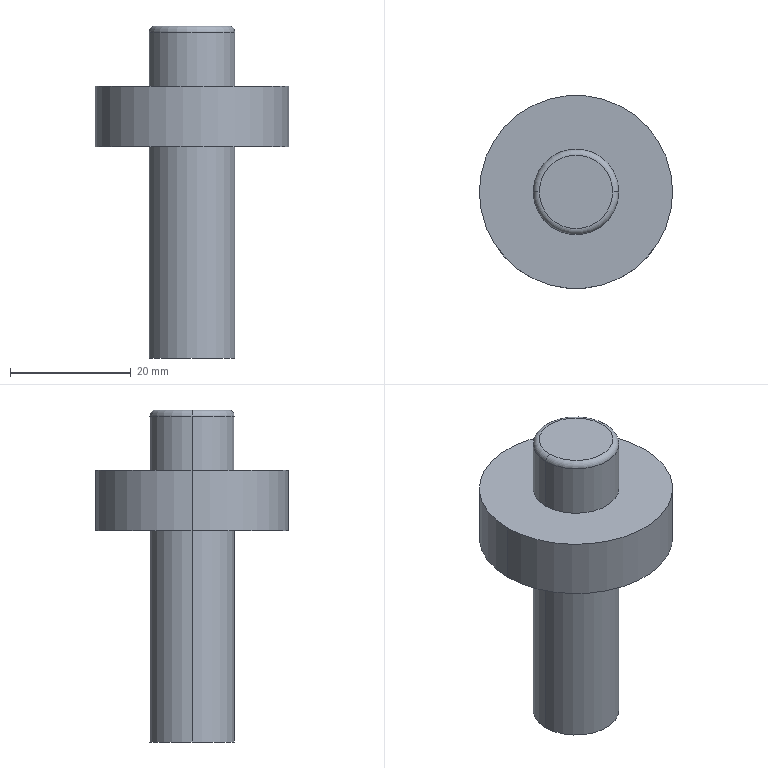Component | SolidWorks | Motor-1 | 1 solid | 12 faces | box 32.01 x 32.01 x 55 mm | volume 15143 mm3 | cylinder 6 | plane 4 | torus 2 | commonest cylinder face diameters 14.18 x4 32.008 x2
build123d program:
from build123d import *

# Parameters (mm, degrees)
SKETCH1_R           = 16.004
BOSS_EXTRUDE1_DEPTH = 10
SKETCH2_R           = 7.09
BOSS_EXTRUDE2_DEPTH = 10
FILLET1_R           = 1
BOSS_EXTRUDE3_START = 35
SKETCH3_R           = 7.09
BOSS_EXTRUDE3_DEPTH = 35


with BuildPart() as part:
    # Sketch1 → Boss-Extrude1 (new body)
    with BuildSketch(Plane.XY):
        with Locations((209.842, -12.569)):
            Circle(SKETCH1_R)
    extrude(amount=BOSS_EXTRUDE1_DEPTH)

    # Sketch2 → Boss-Extrude2 (add)
    with BuildSketch(Plane.XY.offset(10)):
        with Locations((209.842, -12.569)):
            Circle(SKETCH2_R)
    extrude(amount=BOSS_EXTRUDE2_DEPTH)

    # Fillet1
    fillet1_edges = [part.edges().sort_by_distance(p)[0] for p in [
        (202.752, -12.569, 20),
    ]]
    fillet(fillet1_edges, radius=FILLET1_R)

    # Sketch3 → Boss-Extrude3 (add)
    with BuildSketch(Plane(origin=(0, 0, 0), x_dir=(-1, 0, 0), z_dir=(0, 0, -1)).offset(BOSS_EXTRUDE3_START)):
        with Locations(Location((-209.842, -12.569, 0), (0, 0, 180))):
            Circle(SKETCH3_R)
    extrude(amount=-BOSS_EXTRUDE3_DEPTH)


solid = part.part

# Placed as in the assembly
solid = solid.moved(Location((-16.965, 0.5467, 8.5), (0, 0, 0)))
STEP:
#1=COLOUR_RGB('',0.7922,0.8196,0.9333);
#2=FILL_AREA_STYLE_COLOUR('',#1);
#3=FILL_AREA_STYLE('',(#2));
#4=SURFACE_STYLE_FILL_AREA(#3);
#5=SURFACE_SIDE_STYLE('',(#4));
#6=SURFACE_STYLE_USAGE(.BOTH.,#5);
#7=PRESENTATION_STYLE_ASSIGNMENT((#6));
#8=CARTESIAN_POINT('',(7.314,-0.4733,-1.043));
#9=VERTEX_POINT('',#8);
#10=CARTESIAN_POINT('',(7.873,-0.4733,-1.043));
#11=VERTEX_POINT('',#10);
#12=CARTESIAN_POINT('',(7.594,-0.4733,-1.043));
#13=DIRECTION('',(0.,0.,-1.));
#14=DIRECTION('',(-1.,0.,0.));
#15=AXIS2_PLACEMENT_3D('',#12,#13,#14);
#16=CIRCLE('',#15,0.2791);
#17=EDGE_CURVE('',#9,#11,#16,.T.);
#18=ORIENTED_EDGE('',*,*,#17,.F.);
#19=CARTESIAN_POINT('',(7.314,-0.4733,0.3346));
#20=VERTEX_POINT('',#19);
#21=CARTESIAN_POINT('',(7.314,-0.4733,-1.043));
#22=DIRECTION('',(0.,0.,1.));
#23=VECTOR('',#22,39.37);
#24=LINE('',#21,#23);
#25=EDGE_CURVE('',#9,#20,#24,.T.);
#26=ORIENTED_EDGE('',*,*,#25,.T.);
#27=CARTESIAN_POINT('',(7.873,-0.4733,0.3346));
#28=VERTEX_POINT('',#27);
#29=CARTESIAN_POINT('',(7.594,-0.4733,0.3346));
#30=DIRECTION('',(0.,0.,-1.));
#31=DIRECTION('',(-1.,0.,0.));
#32=AXIS2_PLACEMENT_3D('',#29,#30,#31);
#33=CIRCLE('',#32,0.2791);
#34=EDGE_CURVE('',#20,#28,#33,.T.);
#35=ORIENTED_EDGE('',*,*,#34,.T.);
#36=CARTESIAN_POINT('',(7.873,-0.4733,-1.043));
#37=DIRECTION('',(0.,0.,1.));
#38=VECTOR('',#37,39.37);
#39=LINE('',#36,#38);
#40=EDGE_CURVE('',#11,#28,#39,.T.);
#41=ORIENTED_EDGE('',*,*,#40,.F.);
#42=EDGE_LOOP('',(#18,#26,#35,#41));
#43=FACE_OUTER_BOUND('',#42,.T.);
#44=CARTESIAN_POINT('',(7.594,-0.4733,-1.043));
#45=DIRECTION('',(0.,0.,1.));
#46=DIRECTION('',(1.,0.,0.));
#47=AXIS2_PLACEMENT_3D('',#44,#45,#46);
#48=CYLINDRICAL_SURFACE('',#47,0.2791);
#49=ADVANCED_FACE('',(#43),#48,.T.);
#50=CARTESIAN_POINT('',(7.314,-0.4733,1.083));
#51=VERTEX_POINT('',#50);
#52=CARTESIAN_POINT('',(7.873,-0.4733,1.083));
#53=VERTEX_POINT('',#52);
#54=CARTESIAN_POINT('',(7.594,-0.4733,1.083));
#55=DIRECTION('',(0.,0.,-1.));
#56=DIRECTION('',(1.,0.,0.));
#57=AXIS2_PLACEMENT_3D('',#54,#55,#56);
#58=CIRCLE('',#57,0.2791);
#59=EDGE_CURVE('',#51,#53,#58,.T.);
#60=ORIENTED_EDGE('',*,*,#59,.F.);
#61=CARTESIAN_POINT('',(7.354,-0.4733,1.122));
#62=VERTEX_POINT('',#61);
#63=CARTESIAN_POINT('',(7.354,-0.4733,1.083));
#64=DIRECTION('',(0.,1.,0.));
#65=DIRECTION('',(-1.,0.,0.));
#66=AXIS2_PLACEMENT_3D('',#63,#64,#65);
#67=CIRCLE('',#66,0.03937);
#68=EDGE_CURVE('',#51,#62,#67,.T.);
#69=ORIENTED_EDGE('',*,*,#68,.T.);
#70=CARTESIAN_POINT('',(7.833,-0.4733,1.122));
#71=VERTEX_POINT('',#70);
#72=CARTESIAN_POINT('',(7.594,-0.4733,1.122));
#73=DIRECTION('',(0.,0.,1.));
#74=DIRECTION('',(1.,0.,0.));
#75=AXIS2_PLACEMENT_3D('',#72,#73,#74);
#76=CIRCLE('',#75,0.2398);
#77=EDGE_CURVE('',#71,#62,#76,.T.);
#78=ORIENTED_EDGE('',*,*,#77,.F.);
#79=CARTESIAN_POINT('',(7.833,-0.4733,1.083));
#80=DIRECTION('',(0.,-1.,0.));
#81=DIRECTION('',(0.,0.,-1.));
#82=AXIS2_PLACEMENT_3D('',#79,#80,#81);
#83=CIRCLE('',#82,0.03937);
#84=EDGE_CURVE('',#53,#71,#83,.T.);
#85=ORIENTED_EDGE('',*,*,#84,.F.);
#86=EDGE_LOOP('',(#60,#69,#78,#85));
#87=FACE_OUTER_BOUND('',#86,.T.);
#88=CARTESIAN_POINT('',(7.594,-0.4733,1.083));
#89=DIRECTION('',(0.,0.,1.));
#90=DIRECTION('',(1.,0.,0.));
#91=AXIS2_PLACEMENT_3D('',#88,#89,#90);
#92=TOROIDAL_SURFACE('',#91,0.2398,0.03937);
#93=ADVANCED_FACE('',(#87),#92,.T.);
#94=ORIENTED_EDGE('',*,*,#59,.T.);
#95=CARTESIAN_POINT('',(7.873,-0.4733,0.7283));
#96=VERTEX_POINT('',#95);
#97=CARTESIAN_POINT('',(7.873,-0.4733,1.122));
#98=DIRECTION('',(0.,0.,-1.));
#99=VECTOR('',#98,39.37);
#100=LINE('',#97,#99);
#101=EDGE_CURVE('',#53,#96,#100,.T.);
#102=ORIENTED_EDGE('',*,*,#101,.T.);
#103=CARTESIAN_POINT('',(7.314,-0.4733,0.7283));
#104=VERTEX_POINT('',#103);
#105=CARTESIAN_POINT('',(7.594,-0.4733,0.7283));
#106=DIRECTION('',(0.,0.,1.));
#107=DIRECTION('',(1.,0.,0.));
#108=AXIS2_PLACEMENT_3D('',#105,#106,#107);
#109=CIRCLE('',#108,0.2791);
#110=EDGE_CURVE('',#96,#104,#109,.T.);
#111=ORIENTED_EDGE('',*,*,#110,.T.);
#112=CARTESIAN_POINT('',(7.314,-0.4733,1.122));
#113=DIRECTION('',(0.,0.,-1.));
#114=VECTOR('',#113,39.37);
#115=LINE('',#112,#114);
#116=EDGE_CURVE('',#51,#104,#115,.T.);
#117=ORIENTED_EDGE('',*,*,#116,.F.);
#118=EDGE_LOOP('',(#94,#102,#111,#117));
#119=FACE_OUTER_BOUND('',#118,.T.);
#120=CARTESIAN_POINT('',(7.594,-0.4733,1.122));
#121=DIRECTION('',(0.,0.,-1.));
#122=DIRECTION('',(-1.,0.,0.));
#123=AXIS2_PLACEMENT_3D('',#120,#121,#122);
#124=CYLINDRICAL_SURFACE('',#123,0.2791);
#125=ADVANCED_FACE('',(#119),#124,.T.);
#126=CARTESIAN_POINT('',(8.224,-0.4733,0.7283));
#127=VERTEX_POINT('',#126);
#128=CARTESIAN_POINT('',(6.964,-0.4733,0.7283));
#129=VERTEX_POINT('',#128);
#130=CARTESIAN_POINT('',(7.594,-0.4733,0.7283));
#131=DIRECTION('',(0.,0.,1.));
#132=DIRECTION('',(1.,0.,0.));
#133=AXIS2_PLACEMENT_3D('',#130,#131,#132);
#134=CIRCLE('',#133,0.6301);
#135=EDGE_CURVE('',#127,#129,#134,.T.);
#136=ORIENTED_EDGE('',*,*,#135,.F.);
#137=CARTESIAN_POINT('',(8.224,-0.4733,0.3346));
#138=VERTEX_POINT('',#137);
#139=CARTESIAN_POINT('',(8.224,-0.4733,0.7283));
#140=DIRECTION('',(0.,0.,-1.));
#141=VECTOR('',#140,39.37);
#142=LINE('',#139,#141);
#143=EDGE_CURVE('',#127,#138,#142,.T.);
#144=ORIENTED_EDGE('',*,*,#143,.T.);
#145=CARTESIAN_POINT('',(6.964,-0.4733,0.3346));
#146=VERTEX_POINT('',#145);
#147=CARTESIAN_POINT('',(7.594,-0.4733,0.3346));
#148=DIRECTION('',(0.,0.,1.));
#149=DIRECTION('',(1.,0.,0.));
#150=AXIS2_PLACEMENT_3D('',#147,#148,#149);
#151=CIRCLE('',#150,0.6301);
#152=EDGE_CURVE('',#138,#146,#151,.T.);
#153=ORIENTED_EDGE('',*,*,#152,.T.);
#154=CARTESIAN_POINT('',(6.964,-0.4733,0.7283));
#155=DIRECTION('',(0.,0.,-1.));
#156=VECTOR('',#155,39.37);
#157=LINE('',#154,#156);
#158=EDGE_CURVE('',#129,#146,#157,.T.);
#159=ORIENTED_EDGE('',*,*,#158,.F.);
#160=EDGE_LOOP('',(#136,#144,#153,#159));
#161=FACE_OUTER_BOUND('',#160,.T.);
#162=CARTESIAN_POINT('',(7.594,-0.4733,0.7283));
#163=DIRECTION('',(0.,0.,-1.));
#164=DIRECTION('',(-1.,0.,0.));
#165=AXIS2_PLACEMENT_3D('',#162,#163,#164);
#166=CYLINDRICAL_SURFACE('',#165,0.6301);
#167=ADVANCED_FACE('',(#161),#166,.T.);
#168=ORIENTED_EDGE('',*,*,#143,.F.);
#169=CARTESIAN_POINT('',(7.594,-0.4733,0.7283));
#170=DIRECTION('',(0.,0.,1.));
#171=DIRECTION('',(1.,0.,0.));
#172=AXIS2_PLACEMENT_3D('',#169,#170,#171);
#173=CIRCLE('',#172,0.6301);
#174=EDGE_CURVE('',#129,#127,#173,.T.);
#175=ORIENTED_EDGE('',*,*,#174,.F.);
#176=ORIENTED_EDGE('',*,*,#158,.T.);
#177=CARTESIAN_POINT('',(7.594,-0.4733,0.3346));
#178=DIRECTION('',(0.,0.,1.));
#179=DIRECTION('',(1.,0.,0.));
#180=AXIS2_PLACEMENT_3D('',#177,#178,#179);
#181=CIRCLE('',#180,0.6301);
#182=EDGE_CURVE('',#146,#138,#181,.T.);
#183=ORIENTED_EDGE('',*,*,#182,.T.);
#184=EDGE_LOOP('',(#168,#175,#176,#183));
#185=FACE_OUTER_BOUND('',#184,.T.);
#186=CARTESIAN_POINT('',(7.594,-0.4733,0.7283));
#187=DIRECTION('',(0.,0.,-1.));
#188=DIRECTION('',(-1.,0.,0.));
#189=AXIS2_PLACEMENT_3D('',#186,#187,#188);
#190=CYLINDRICAL_SURFACE('',#189,0.6301);
#191=ADVANCED_FACE('',(#185),#190,.T.);
#192=CARTESIAN_POINT('',(7.594,-0.4733,0.7283));
#193=DIRECTION('',(0.,0.,1.));
#194=DIRECTION('',(1.,0.,0.));
#195=AXIS2_PLACEMENT_3D('',#192,#193,#194);
#196=CIRCLE('',#195,0.2791);
#197=EDGE_CURVE('',#104,#96,#196,.T.);
#198=ORIENTED_EDGE('',*,*,#197,.F.);
#199=ORIENTED_EDGE('',*,*,#110,.F.);
#200=EDGE_LOOP('',(#198,#199));
#201=FACE_BOUND('',#200,.T.);
#202=ORIENTED_EDGE('',*,*,#174,.T.);
#203=ORIENTED_EDGE('',*,*,#135,.T.);
#204=EDGE_LOOP('',(#202,#203));
#205=FACE_OUTER_BOUND('',#204,.T.);
#206=CARTESIAN_POINT('',(7.594,-0.4733,0.7283));
#207=DIRECTION('',(0.,0.,1.));
#208=DIRECTION('',(1.,0.,0.));
#209=AXIS2_PLACEMENT_3D('',#206,#207,#208);
#210=PLANE('',#209);
#211=ADVANCED_FACE('',(#201,#205),#210,.T.);
#212=CARTESIAN_POINT('',(7.594,-0.4733,0.3346));
#213=DIRECTION('',(0.,0.,-1.));
#214=DIRECTION('',(-1.,0.,0.));
#215=AXIS2_PLACEMENT_3D('',#212,#213,#214);
#216=CIRCLE('',#215,0.2791);
#217=EDGE_CURVE('',#28,#20,#216,.T.);
#218=ORIENTED_EDGE('',*,*,#217,.F.);
#219=ORIENTED_EDGE('',*,*,#34,.F.);
#220=EDGE_LOOP('',(#218,#219));
#221=FACE_BOUND('',#220,.T.);
#222=ORIENTED_EDGE('',*,*,#182,.F.);
#223=ORIENTED_EDGE('',*,*,#152,.F.);
#224=EDGE_LOOP('',(#222,#223));
#225=FACE_OUTER_BOUND('',#224,.T.);
#226=CARTESIAN_POINT('',(7.594,-0.4733,0.3346));
#227=DIRECTION('',(0.,0.,1.));
#228=DIRECTION('',(1.,0.,0.));
#229=AXIS2_PLACEMENT_3D('',#226,#227,#228);
#230=PLANE('',#229);
#231=ADVANCED_FACE('',(#221,#225),#230,.F.);
#232=ORIENTED_EDGE('',*,*,#101,.F.);
#233=CARTESIAN_POINT('',(7.594,-0.4733,1.083));
#234=DIRECTION('',(0.,0.,-1.));
#235=DIRECTION('',(1.,0.,0.));
#236=AXIS2_PLACEMENT_3D('',#233,#234,#235);
#237=CIRCLE('',#236,0.2791);
#238=EDGE_CURVE('',#53,#51,#237,.T.);
#239=ORIENTED_EDGE('',*,*,#238,.T.);
#240=ORIENTED_EDGE('',*,*,#116,.T.);
#241=ORIENTED_EDGE('',*,*,#197,.T.);
#242=EDGE_LOOP('',(#232,#239,#240,#241));
#243=FACE_OUTER_BOUND('',#242,.T.);
#244=CARTESIAN_POINT('',(7.594,-0.4733,1.122));
#245=DIRECTION('',(0.,0.,-1.));
#246=DIRECTION('',(-1.,0.,0.));
#247=AXIS2_PLACEMENT_3D('',#244,#245,#246);
#248=CYLINDRICAL_SURFACE('',#247,0.2791);
#249=ADVANCED_FACE('',(#243),#248,.T.);
#250=ORIENTED_EDGE('',*,*,#77,.T.);
#251=CARTESIAN_POINT('',(7.594,-0.4733,1.122));
#252=DIRECTION('',(0.,0.,1.));
#253=DIRECTION('',(1.,0.,0.));
#254=AXIS2_PLACEMENT_3D('',#251,#252,#253);
#255=CIRCLE('',#254,0.2398);
#256=EDGE_CURVE('',#62,#71,#255,.T.);
#257=ORIENTED_EDGE('',*,*,#256,.T.);
#258=EDGE_LOOP('',(#250,#257));
#259=FACE_OUTER_BOUND('',#258,.T.);
#260=CARTESIAN_POINT('',(7.594,-0.4733,1.122));
#261=DIRECTION('',(0.,0.,1.));
#262=DIRECTION('',(1.,0.,0.));
#263=AXIS2_PLACEMENT_3D('',#260,#261,#262);
#264=PLANE('',#263);
#265=ADVANCED_FACE('',(#259),#264,.T.);
#266=ORIENTED_EDGE('',*,*,#68,.F.);
#267=ORIENTED_EDGE('',*,*,#238,.F.);
#268=ORIENTED_EDGE('',*,*,#84,.T.);
#269=ORIENTED_EDGE('',*,*,#256,.F.);
#270=EDGE_LOOP('',(#266,#267,#268,#269));
#271=FACE_OUTER_BOUND('',#270,.T.);
#272=CARTESIAN_POINT('',(7.594,-0.4733,1.083));
#273=DIRECTION('',(0.,0.,1.));
#274=DIRECTION('',(1.,0.,0.));
#275=AXIS2_PLACEMENT_3D('',#272,#273,#274);
#276=TOROIDAL_SURFACE('',#275,0.2398,0.03937);
#277=ADVANCED_FACE('',(#271),#276,.T.);
#278=ORIENTED_EDGE('',*,*,#25,.F.);
#279=CARTESIAN_POINT('',(7.594,-0.4733,-1.043));
#280=DIRECTION('',(0.,0.,-1.));
#281=DIRECTION('',(-1.,0.,0.));
#282=AXIS2_PLACEMENT_3D('',#279,#280,#281);
#283=CIRCLE('',#282,0.2791);
#284=EDGE_CURVE('',#11,#9,#283,.T.);
#285=ORIENTED_EDGE('',*,*,#284,.F.);
#286=ORIENTED_EDGE('',*,*,#40,.T.);
#287=ORIENTED_EDGE('',*,*,#217,.T.);
#288=EDGE_LOOP('',(#278,#285,#286,#287));
#289=FACE_OUTER_BOUND('',#288,.T.);
#290=CARTESIAN_POINT('',(7.594,-0.4733,-1.043));
#291=DIRECTION('',(0.,0.,1.));
#292=DIRECTION('',(1.,0.,0.));
#293=AXIS2_PLACEMENT_3D('',#290,#291,#292);
#294=CYLINDRICAL_SURFACE('',#293,0.2791);
#295=ADVANCED_FACE('',(#289),#294,.T.);
#296=ORIENTED_EDGE('',*,*,#284,.T.);
#297=ORIENTED_EDGE('',*,*,#17,.T.);
#298=EDGE_LOOP('',(#296,#297));
#299=FACE_OUTER_BOUND('',#298,.T.);
#300=CARTESIAN_POINT('',(7.594,-0.4733,-1.043));
#301=DIRECTION('',(0.,0.,-1.));
#302=DIRECTION('',(-1.,0.,0.));
#303=AXIS2_PLACEMENT_3D('',#300,#301,#302);
#304=PLANE('',#303);
#305=ADVANCED_FACE('',(#299),#304,.T.);
#306=CLOSED_SHELL('',(#49,#93,#125,#167,#191,#211,#231,#249,#265,#277,#295,#305));
#307=MANIFOLD_SOLID_BREP('',#306);
#308=STYLED_ITEM('',(#7),#307);
#309=(LENGTH_UNIT()NAMED_UNIT(*)SI_UNIT($,.METRE.));
#310=LENGTH_MEASURE_WITH_UNIT(LENGTH_MEASURE(0.0254),#309);
#311=DIMENSIONAL_EXPONENTS(1.,0.,0.,0.,0.,0.,0.);
#312=(CONVERSION_BASED_UNIT('',#310)LENGTH_UNIT()NAMED_UNIT(#311));
#313=UNCERTAINTY_MEASURE_WITH_UNIT(LENGTH_MEASURE(0.00001),#312,'','');
#314=(NAMED_UNIT(*)PLANE_ANGLE_UNIT()SI_UNIT($,.RADIAN.));
#315=(NAMED_UNIT(*)SI_UNIT($,.STERADIAN.)SOLID_ANGLE_UNIT());
#316=(GEOMETRIC_REPRESENTATION_CONTEXT(3)GLOBAL_UNCERTAINTY_ASSIGNED_CONTEXT((#313))GLOBAL_UNIT_ASSIGNED_CONTEXT((#312,#314,#315))REPRESENTATION_CONTEXT('',''));
#317=MECHANICAL_DESIGN_GEOMETRIC_PRESENTATION_REPRESENTATION('',(#308),#316);
#318=CARTESIAN_POINT('',(0.,0.,0.));
#319=DIRECTION('',(0.,0.,1.));
#320=DIRECTION('',(1.,0.,0.));
#321=AXIS2_PLACEMENT_3D('',#318,#319,#320);
#322=(LENGTH_UNIT()NAMED_UNIT(*)SI_UNIT($,.METRE.));
#323=LENGTH_MEASURE_WITH_UNIT(LENGTH_MEASURE(0.0254),#322);
#324=DIMENSIONAL_EXPONENTS(1.,0.,0.,0.,0.,0.,0.);
#325=(CONVERSION_BASED_UNIT('',#323)LENGTH_UNIT()NAMED_UNIT(#324));
#326=UNCERTAINTY_MEASURE_WITH_UNIT(LENGTH_MEASURE(0.00001),#325,'','');
#327=(NAMED_UNIT(*)PLANE_ANGLE_UNIT()SI_UNIT($,.RADIAN.));
#328=(NAMED_UNIT(*)SI_UNIT($,.STERADIAN.)SOLID_ANGLE_UNIT());
#329=(GEOMETRIC_REPRESENTATION_CONTEXT(3)GLOBAL_UNCERTAINTY_ASSIGNED_CONTEXT((#326))GLOBAL_UNIT_ASSIGNED_CONTEXT((#325,#327,#328))REPRESENTATION_CONTEXT('',''));
#330=ADVANCED_BREP_SHAPE_REPRESENTATION('',(#307,#321),#329);
#331=PRESENTATION_LAYER_ASSIGNMENT('','',(#308));